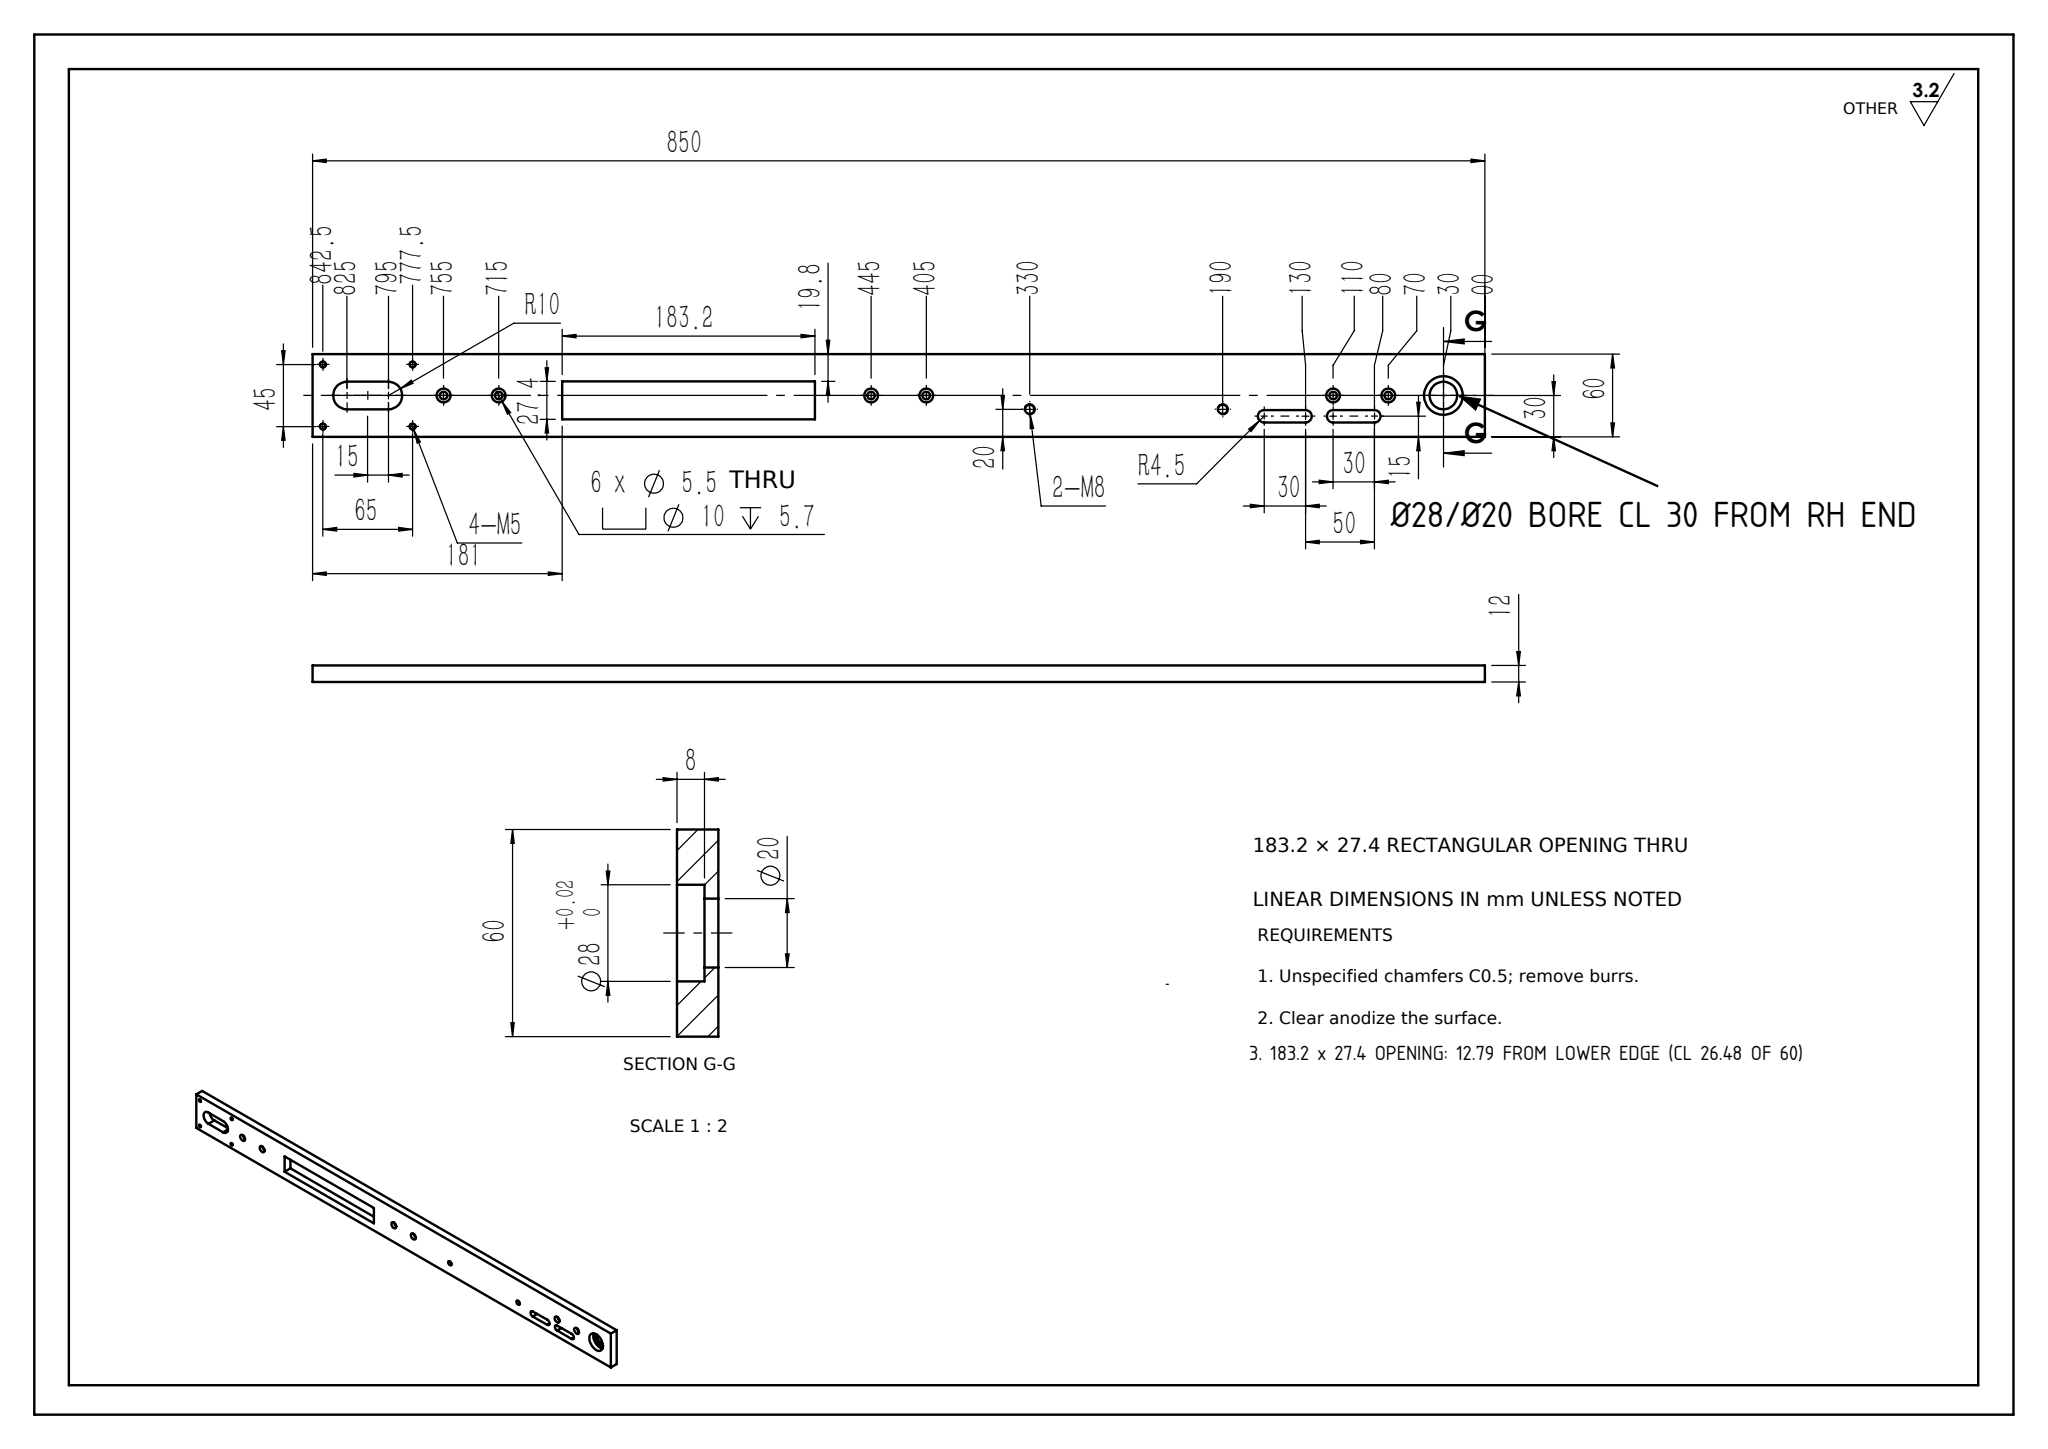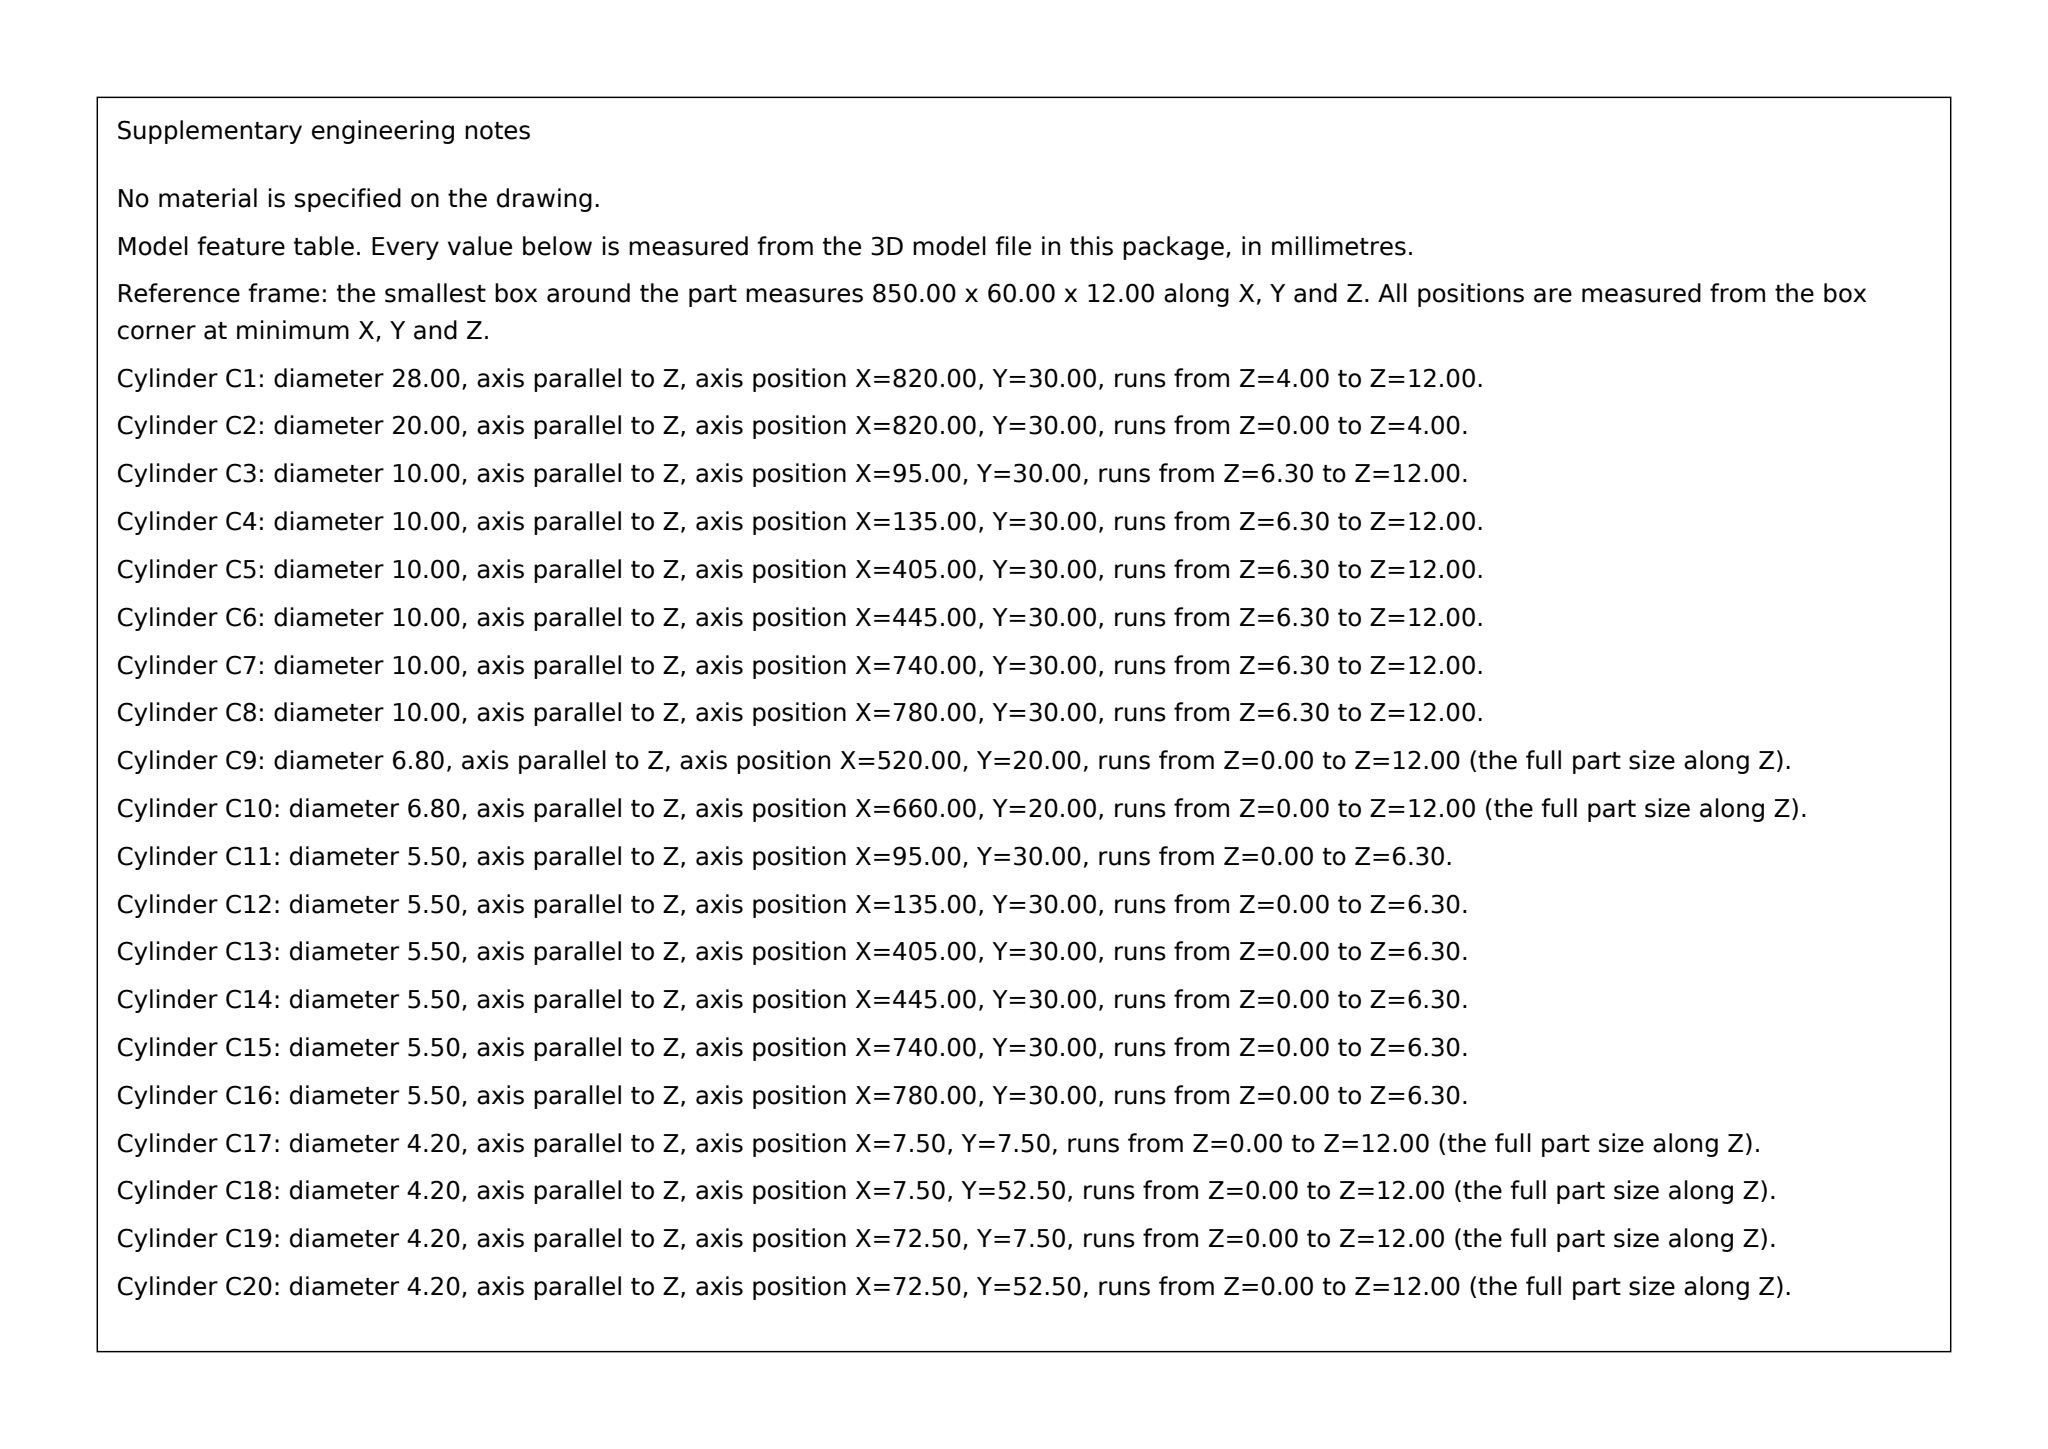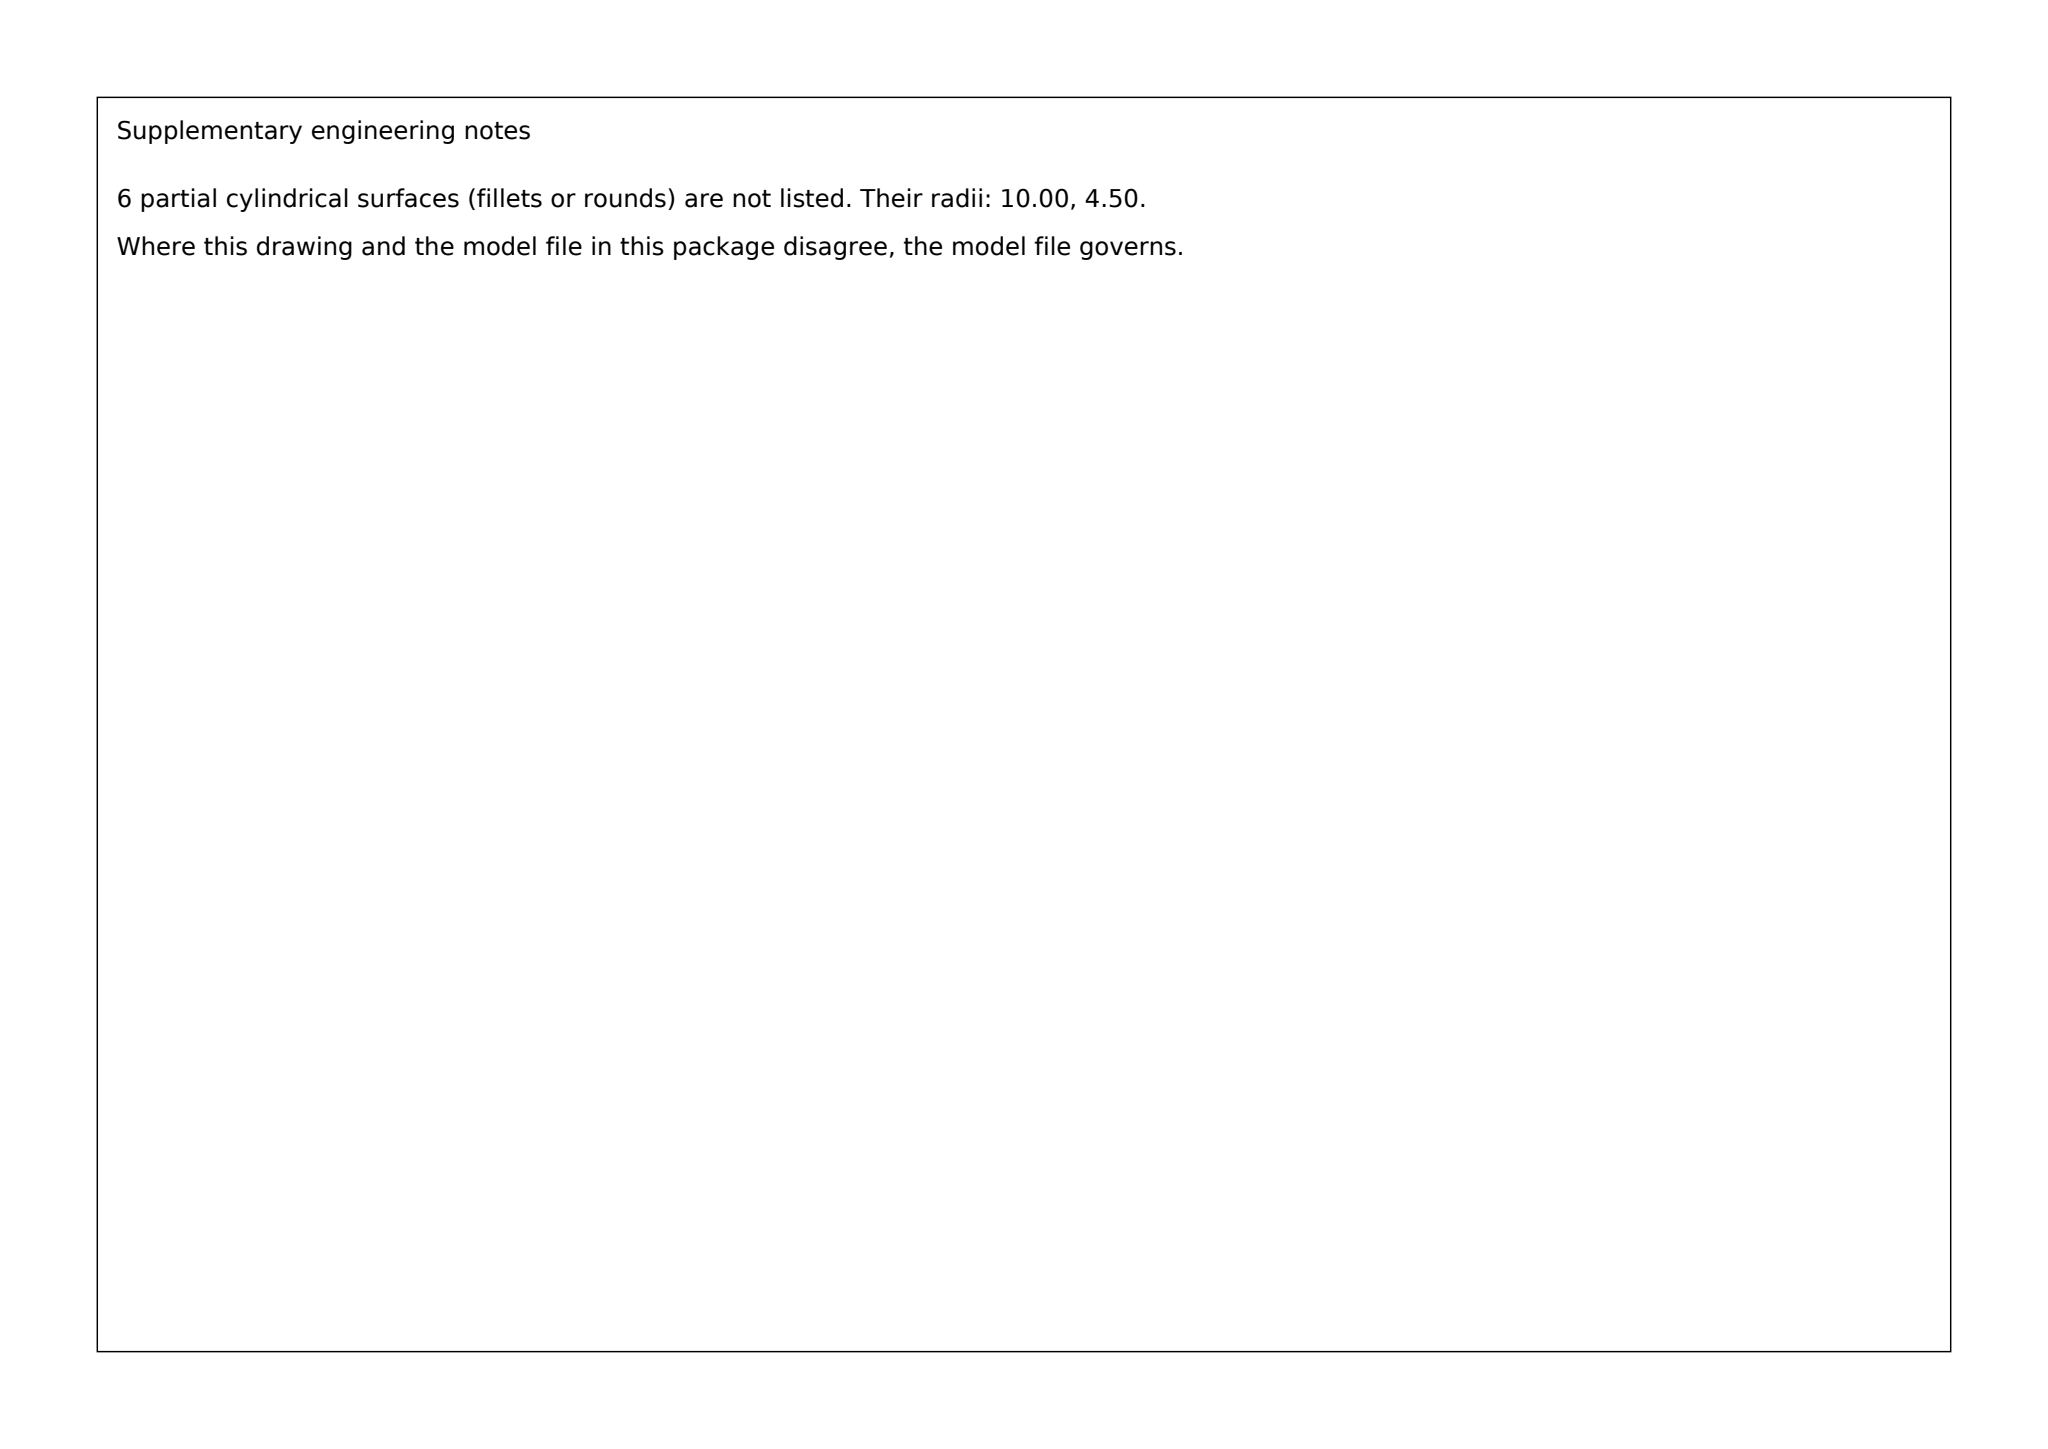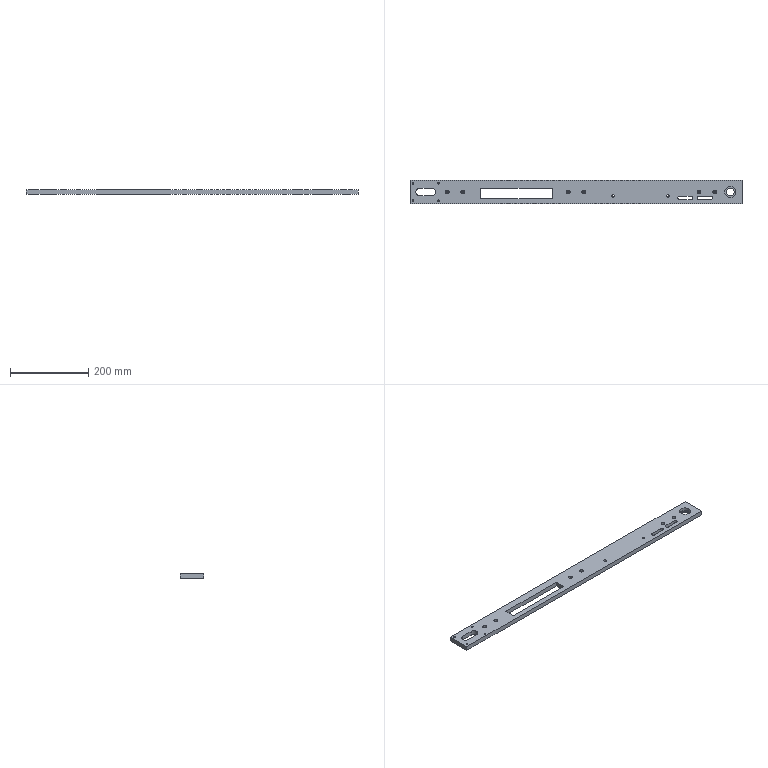Part | SolidWorks | mm | 1 solid | 72 faces | box 850 x 60 x 12 mm | volume 521520 mm3 | cylinder 49 | plane 23 | commonest cylinder face diameters 10 x12 5.5 x12 4.2 x8 9 x6 20 x5 6.8 x4 28 x2
Drawing notes:
183.2 x 27.4 OPENING: 12.79 FROM LOWER EDGE (CL 26.48 OF 60) | from the solid: y-planes 12.79 and 40.17 bound the 27.4 opening; part width y 0 to 60
ORDINATE ZERO AT RH END FACE; Ø28/Ø20 BORE CL 30 FROM RH END | from the solid: bbox x=850 RH face; Ø28 & Ø20 bores axis at x=820, y=30 => 850-820=30; ordinate labels 842.5/825/.../30 all = 850-x
build123d program:
from build123d import *

# Parameters (mm, degrees)
SKETCH1_W                                            = 850
SKETCH1_H                                            = 60
BOSS_EXTRUDE1_DEPTH                                  = 12
SKETCH2_R                                            = 10
CUT_EXTRUDE1_DEPTH                                   = 427.226
SKETCH3_R                                            = 14
CUT_EXTRUDE2_DEPTH                                   = 8
M5_TAPPED_HOLE1_D                                    = 4.2
M5_TAPPED_HOLE1_DEPTH                                = 12.4
M5_TAPPED_HOLE1_TIP                                  = 1.262
CUT_EXTRUDE3_DEPTH                                   = 427.226
HOLE_SIZE_ACCORDING_TO_HEX_SOCKET_HEAD_C_D           = 5.5
HOLE_SIZE_ACCORDING_TO_HEX_SOCKET_HEAD_C_CBORE_D     = 10
HOLE_SIZE_ACCORDING_TO_HEX_SOCKET_HEAD_C_CBORE_DEPTH = 5.7
M8_TAPPED_HOLE1_D                                    = 6.8
M8_TAPPED_HOLE1_DEPTH                                = 19.75
M8_TAPPED_HOLE1_TIP                                  = 2.043
SKETCH13_W                                           = 183.243
SKETCH13_H                                           = 27.377
CUT_EXTRUDE4_DEPTH                                   = 340


with BuildPart() as part:
    # Sketch1 → Boss-Extrude1 (new body)
    with BuildSketch(Plane.XY):
        Rectangle(SKETCH1_W, SKETCH1_H)
    extrude(amount=BOSS_EXTRUDE1_DEPTH)

    # Sketch2 → Cut-Extrude1 (cut, through all)
    with BuildSketch(Plane.XY.offset(12)):
        with Locations((395, 0)):
            Circle(SKETCH2_R)
        with BuildLine():
            Line((-400, 10), (-370, 10))
            ThreePointArc((-370, 10), (-360, 0), (-370, -10))
            Line((-370, -10), (-400, -10))
            ThreePointArc((-400, -10), (-410, 0), (-400, 10))
        make_face()
    extrude(amount=-CUT_EXTRUDE1_DEPTH, mode=Mode.SUBTRACT)

    # Sketch3 → Cut-Extrude2 (cut)
    with BuildSketch(Plane.XY.offset(12)):
        with Locations((395, 0)):
            Circle(SKETCH3_R)
    extrude(amount=-CUT_EXTRUDE2_DEPTH, mode=Mode.SUBTRACT)

    # M5 Tapped Hole1
    with Locations(Plane.XY.offset(12)):
        with Locations((-417.5, -22.5), (-352.5, -22.5), (-352.5, 22.5), (-417.5, 22.5)):
            Hole(M5_TAPPED_HOLE1_D / 2, depth=M5_TAPPED_HOLE1_DEPTH)
            with Locations((0, 0, -(M5_TAPPED_HOLE1_DEPTH + M5_TAPPED_HOLE1_TIP / 2))):  # 118° drill point
                Cone(0, M5_TAPPED_HOLE1_D / 2, M5_TAPPED_HOLE1_TIP, mode=Mode.SUBTRACT)

    # Sketch8 → Cut-Extrude3 (cut, through all)
    with BuildSketch(Plane.XY.offset(12)):
        with BuildLine():
            Line((315, -10.5), (345, -10.5))
            ThreePointArc((345, -10.5), (349.5, -15), (345, -19.5))
            Line((345, -19.5), (315, -19.5))
            ThreePointArc((315, -19.5), (310.5, -15), (315, -10.5))
        make_face()
        with BuildLine():
            Line((295, -19.5), (265, -19.5))
            ThreePointArc((265, -19.5), (260.5, -15), (265, -10.5))
            Line((265, -10.5), (295, -10.5))
            ThreePointArc((295, -10.5), (299.5, -15), (295, -19.5))
        make_face()
    extrude(amount=-CUT_EXTRUDE3_DEPTH, mode=Mode.SUBTRACT)

    # Hole Size according to Hex Socket Head C (through all)
    with Locations(Plane.XY.offset(12)):
        with Locations((-330, 0), (-290, 0), (-20, 0), (20, 0), (355, 0), (315, 0)):
            CounterBoreHole(HOLE_SIZE_ACCORDING_TO_HEX_SOCKET_HEAD_C_D / 2, HOLE_SIZE_ACCORDING_TO_HEX_SOCKET_HEAD_C_CBORE_D / 2, HOLE_SIZE_ACCORDING_TO_HEX_SOCKET_HEAD_C_CBORE_DEPTH)

    # M8 Tapped Hole1
    with Locations(Plane.XY.offset(12)):
        with Locations((235, -10), (95, -10)):
            Hole(M8_TAPPED_HOLE1_D / 2, depth=M8_TAPPED_HOLE1_DEPTH)
            with Locations((0, 0, -(M8_TAPPED_HOLE1_DEPTH + M8_TAPPED_HOLE1_TIP / 2))):  # 118° drill point
                Cone(0, M8_TAPPED_HOLE1_D / 2, M8_TAPPED_HOLE1_TIP, mode=Mode.SUBTRACT)

    # Sketch13 → Cut-Extrude4 (cut)
    with BuildSketch(Plane.XY.offset(12)):
        with Locations((-152.367, -3.523)):
            Rectangle(SKETCH13_W, SKETCH13_H)
    extrude(amount=-CUT_EXTRUDE4_DEPTH, mode=Mode.SUBTRACT)


solid = part.part